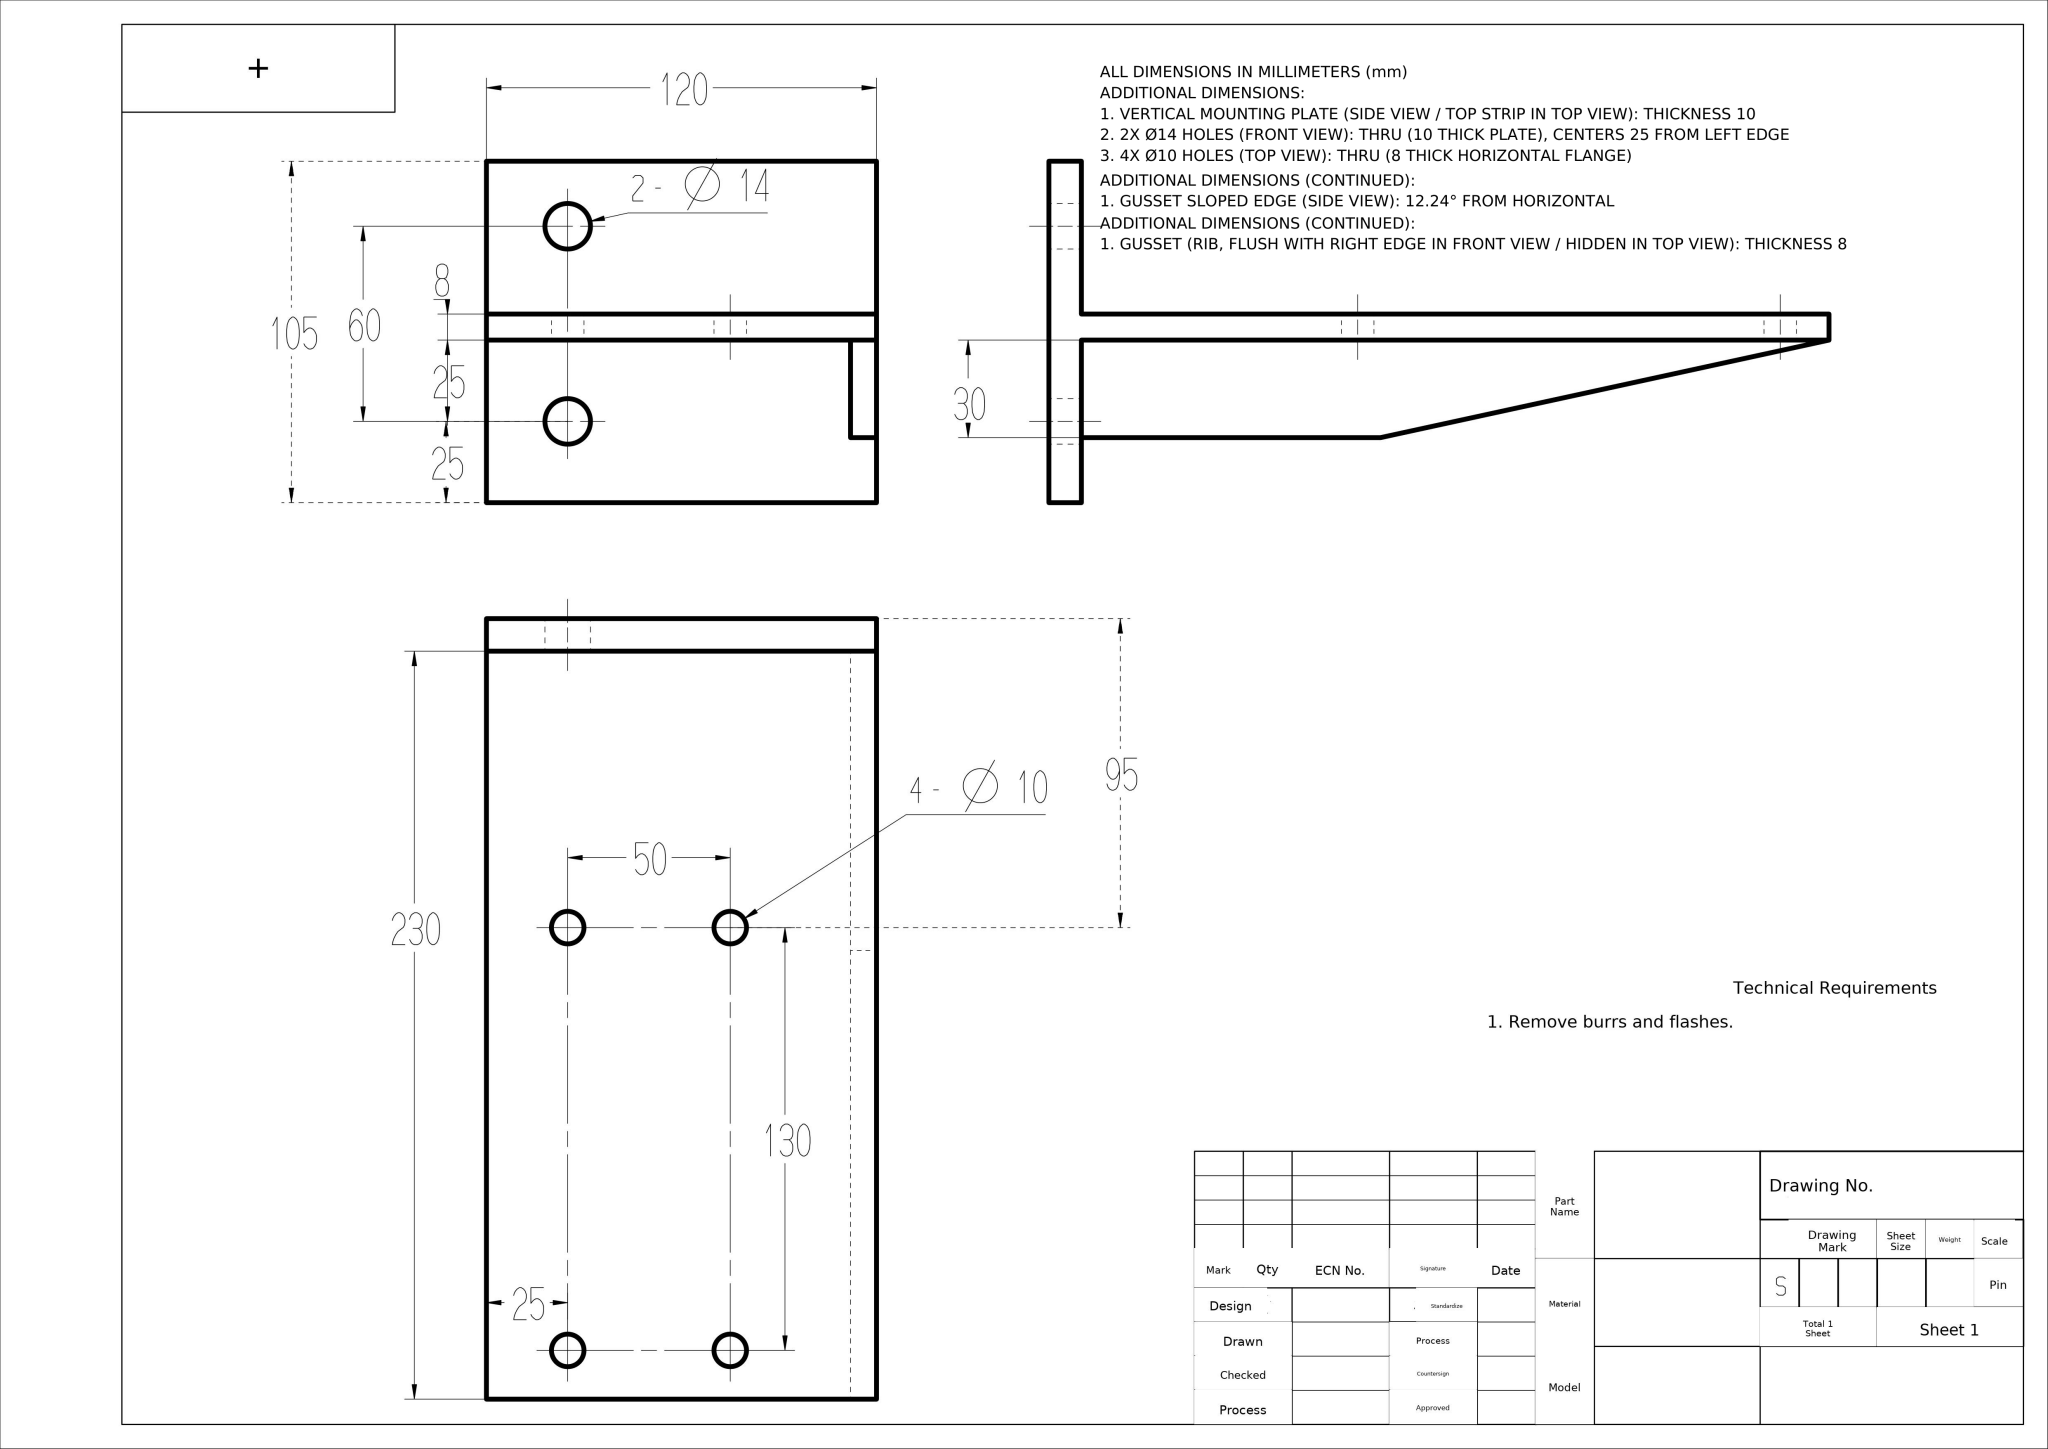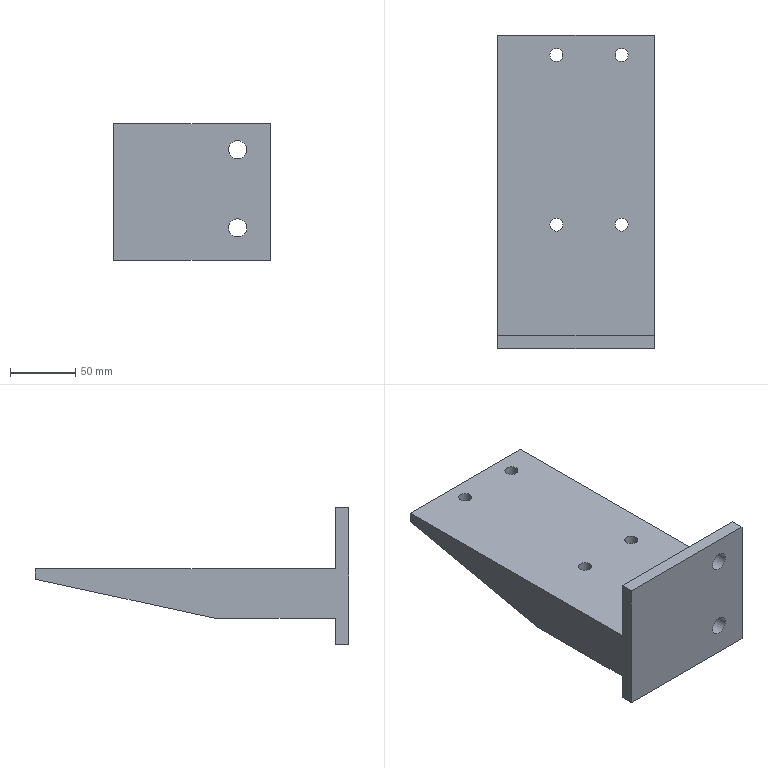Part | NX | mm | 1 solid | 19 faces | box 120 x 240 x 105 mm | volume 379848 mm3 | plane 13 | cylinder 6 | commonest cylinder face diameters 10 x4 14 x2
STEP:
#1=CARTESIAN_POINT('',(0.,0.,0.));
#2=DIRECTION('',(0.,0.,1.));
#3=DIRECTION('',(1.,0.,0.));
#4=AXIS2_PLACEMENT_3D('',#1,#2,#3);
#5=(LENGTH_UNIT()NAMED_UNIT(*)SI_UNIT(.MILLI.,.METRE.));
#6=UNCERTAINTY_MEASURE_WITH_UNIT(LENGTH_MEASURE(0.00002),#5,'','');
#7=(NAMED_UNIT(*)PLANE_ANGLE_UNIT()SI_UNIT($,.RADIAN.));
#8=PLANE_ANGLE_MEASURE_WITH_UNIT(PLANE_ANGLE_MEASURE(0.01745),#7);
#9=DIMENSIONAL_EXPONENTS(0.,0.,0.,0.,0.,0.,0.);
#10=(CONVERSION_BASED_UNIT('',#8)NAMED_UNIT(#9)PLANE_ANGLE_UNIT());
#11=(NAMED_UNIT(*)SI_UNIT($,.STERADIAN.)SOLID_ANGLE_UNIT());
#12=(GEOMETRIC_REPRESENTATION_CONTEXT(3)GLOBAL_UNCERTAINTY_ASSIGNED_CONTEXT((#6))GLOBAL_UNIT_ASSIGNED_CONTEXT((#5,#10,#11))REPRESENTATION_CONTEXT('',''));
#13=SHAPE_REPRESENTATION('',(#4),#12);
#14=CARTESIAN_POINT('',(48.,-142.1,0.));
#15=VERTEX_POINT('',#14);
#16=CARTESIAN_POINT('',(43.,-142.1,0.));
#17=DIRECTION('',(0.,0.,-1.));
#18=DIRECTION('',(1.,0.,0.));
#19=AXIS2_PLACEMENT_3D('',#16,#17,#18);
#20=CIRCLE('',#19,5.);
#21=EDGE_CURVE('',#15,#15,#20,.T.);
#22=ORIENTED_EDGE('',*,*,#21,.F.);
#23=EDGE_LOOP('',(#22));
#24=FACE_BOUND('',#23,.T.);
#25=CARTESIAN_POINT('',(48.,-12.1,0.));
#26=VERTEX_POINT('',#25);
#27=CARTESIAN_POINT('',(43.,-12.1,0.));
#28=DIRECTION('',(0.,0.,1.));
#29=DIRECTION('',(1.,0.,0.));
#30=AXIS2_PLACEMENT_3D('',#27,#28,#29);
#31=CIRCLE('',#30,5.);
#32=EDGE_CURVE('',#26,#26,#31,.T.);
#33=ORIENTED_EDGE('',*,*,#32,.T.);
#34=EDGE_LOOP('',(#33));
#35=FACE_BOUND('',#34,.T.);
#36=CARTESIAN_POINT('',(98.,-142.1,0.));
#37=VERTEX_POINT('',#36);
#38=CARTESIAN_POINT('',(93.,-142.1,0.));
#39=DIRECTION('',(0.,0.,1.));
#40=DIRECTION('',(1.,0.,0.));
#41=AXIS2_PLACEMENT_3D('',#38,#39,#40);
#42=CIRCLE('',#41,5.);
#43=EDGE_CURVE('',#37,#37,#42,.T.);
#44=ORIENTED_EDGE('',*,*,#43,.T.);
#45=EDGE_LOOP('',(#44));
#46=FACE_BOUND('',#45,.T.);
#47=CARTESIAN_POINT('',(98.,-12.1,0.));
#48=VERTEX_POINT('',#47);
#49=CARTESIAN_POINT('',(93.,-12.1,0.));
#50=DIRECTION('',(0.,0.,1.));
#51=DIRECTION('',(1.,0.,0.));
#52=AXIS2_PLACEMENT_3D('',#49,#50,#51);
#53=CIRCLE('',#52,5.);
#54=EDGE_CURVE('',#48,#48,#53,.T.);
#55=ORIENTED_EDGE('',*,*,#54,.T.);
#56=EDGE_LOOP('',(#55));
#57=FACE_BOUND('',#56,.T.);
#58=CARTESIAN_POINT('',(118.,-227.1,0.));
#59=VERTEX_POINT('',#58);
#60=CARTESIAN_POINT('',(6.,-227.1,0.));
#61=VERTEX_POINT('',#60);
#62=CARTESIAN_POINT('',(118.,-227.1,0.));
#63=DIRECTION('',(-1.,-0.,0.));
#64=VECTOR('',#63,1.);
#65=LINE('',#62,#64);
#66=EDGE_CURVE('',#59,#61,#65,.T.);
#67=ORIENTED_EDGE('',*,*,#66,.T.);
#68=CARTESIAN_POINT('',(6.,2.9,0.));
#69=VERTEX_POINT('',#68);
#70=CARTESIAN_POINT('',(6.,-227.1,0.));
#71=DIRECTION('',(0.,1.,0.));
#72=VECTOR('',#71,1.);
#73=LINE('',#70,#72);
#74=EDGE_CURVE('',#61,#69,#73,.T.);
#75=ORIENTED_EDGE('',*,*,#74,.T.);
#76=CARTESIAN_POINT('',(118.,2.9,0.));
#77=VERTEX_POINT('',#76);
#78=CARTESIAN_POINT('',(-2.,2.9,0.));
#79=DIRECTION('',(1.,-0.,0.));
#80=VECTOR('',#79,1.);
#81=LINE('',#78,#80);
#82=EDGE_CURVE('',#69,#77,#81,.T.);
#83=ORIENTED_EDGE('',*,*,#82,.T.);
#84=CARTESIAN_POINT('',(118.,2.9,0.));
#85=DIRECTION('',(0.,-1.,0.));
#86=VECTOR('',#85,1.);
#87=LINE('',#84,#86);
#88=EDGE_CURVE('',#77,#59,#87,.T.);
#89=ORIENTED_EDGE('',*,*,#88,.T.);
#90=EDGE_LOOP('',(#67,#75,#83,#89));
#91=FACE_BOUND('',#90,.T.);
#92=CARTESIAN_POINT('',(0.,0.,0.));
#93=DIRECTION('',(0.,0.,-1.));
#94=DIRECTION('',(-1.,0.,0.));
#95=AXIS2_PLACEMENT_3D('',#92,#93,#94);
#96=PLANE('',#95);
#97=ADVANCED_FACE('',(#24,#35,#46,#57,#91),#96,.T.);
#98=CARTESIAN_POINT('',(-2.,2.9,0.));
#99=VERTEX_POINT('',#98);
#100=CARTESIAN_POINT('',(-2.,2.9,0.));
#101=DIRECTION('',(1.,-0.,0.));
#102=VECTOR('',#101,1.);
#103=LINE('',#100,#102);
#104=EDGE_CURVE('',#99,#69,#103,.T.);
#105=ORIENTED_EDGE('',*,*,#104,.F.);
#106=CARTESIAN_POINT('',(-2.,2.9,8.));
#107=VERTEX_POINT('',#106);
#108=CARTESIAN_POINT('',(-2.,2.9,8.));
#109=DIRECTION('',(0.,0.,-1.));
#110=VECTOR('',#109,1.);
#111=LINE('',#108,#110);
#112=EDGE_CURVE('',#107,#99,#111,.T.);
#113=ORIENTED_EDGE('',*,*,#112,.F.);
#114=CARTESIAN_POINT('',(118.,2.9,8.));
#115=VERTEX_POINT('',#114);
#116=CARTESIAN_POINT('',(-2.,2.9,8.));
#117=DIRECTION('',(1.,-0.,0.));
#118=VECTOR('',#117,1.);
#119=LINE('',#116,#118);
#120=EDGE_CURVE('',#107,#115,#119,.T.);
#121=ORIENTED_EDGE('',*,*,#120,.T.);
#122=CARTESIAN_POINT('',(118.,2.9,8.));
#123=DIRECTION('',(0.,0.,-1.));
#124=VECTOR('',#123,1.);
#125=LINE('',#122,#124);
#126=EDGE_CURVE('',#115,#77,#125,.T.);
#127=ORIENTED_EDGE('',*,*,#126,.T.);
#128=ORIENTED_EDGE('',*,*,#82,.F.);
#129=EDGE_LOOP('',(#105,#113,#121,#127,#128));
#130=FACE_OUTER_BOUND('',#129,.T.);
#131=CARTESIAN_POINT('',(-2.,2.9,8.));
#132=DIRECTION('',(0.,1.,0.));
#133=DIRECTION('',(-1.,0.,0.));
#134=AXIS2_PLACEMENT_3D('',#131,#132,#133);
#135=PLANE('',#134);
#136=ADVANCED_FACE('',(#130),#135,.T.);
#137=ORIENTED_EDGE('',*,*,#88,.F.);
#138=ORIENTED_EDGE('',*,*,#126,.F.);
#139=CARTESIAN_POINT('',(118.,-227.1,8.));
#140=VERTEX_POINT('',#139);
#141=CARTESIAN_POINT('',(118.,2.9,8.));
#142=DIRECTION('',(0.,-1.,0.));
#143=VECTOR('',#142,1.);
#144=LINE('',#141,#143);
#145=EDGE_CURVE('',#115,#140,#144,.T.);
#146=ORIENTED_EDGE('',*,*,#145,.T.);
#147=CARTESIAN_POINT('',(118.,-227.1,55.));
#148=VERTEX_POINT('',#147);
#149=CARTESIAN_POINT('',(118.,-227.1,55.));
#150=DIRECTION('',(0.,0.,1.));
#151=VECTOR('',#150,1.);
#152=LINE('',#149,#151);
#153=EDGE_CURVE('',#140,#148,#152,.T.);
#154=ORIENTED_EDGE('',*,*,#153,.T.);
#155=CARTESIAN_POINT('',(118.,-237.1,55.));
#156=VERTEX_POINT('',#155);
#157=CARTESIAN_POINT('',(118.,-237.1,55.));
#158=DIRECTION('',(0.,-1.,0.));
#159=VECTOR('',#158,1.);
#160=LINE('',#157,#159);
#161=EDGE_CURVE('',#148,#156,#160,.T.);
#162=ORIENTED_EDGE('',*,*,#161,.T.);
#163=CARTESIAN_POINT('',(118.,-237.1,-50.));
#164=VERTEX_POINT('',#163);
#165=CARTESIAN_POINT('',(118.,-237.1,55.));
#166=DIRECTION('',(0.,0.,1.));
#167=VECTOR('',#166,1.);
#168=LINE('',#165,#167);
#169=EDGE_CURVE('',#164,#156,#168,.T.);
#170=ORIENTED_EDGE('',*,*,#169,.F.);
#171=CARTESIAN_POINT('',(118.,-227.1,-50.));
#172=VERTEX_POINT('',#171);
#173=CARTESIAN_POINT('',(118.,-237.1,-50.));
#174=DIRECTION('',(0.,-1.,0.));
#175=VECTOR('',#174,1.);
#176=LINE('',#173,#175);
#177=EDGE_CURVE('',#172,#164,#176,.T.);
#178=ORIENTED_EDGE('',*,*,#177,.F.);
#179=CARTESIAN_POINT('',(118.,-227.1,55.));
#180=DIRECTION('',(0.,0.,1.));
#181=VECTOR('',#180,1.);
#182=LINE('',#179,#181);
#183=EDGE_CURVE('',#172,#59,#182,.T.);
#184=ORIENTED_EDGE('',*,*,#183,.T.);
#185=EDGE_LOOP('',(#137,#138,#146,#154,#162,#170,#178,#184));
#186=FACE_OUTER_BOUND('',#185,.T.);
#187=CARTESIAN_POINT('',(118.,2.9,8.));
#188=DIRECTION('',(1.,0.,0.));
#189=DIRECTION('',(0.,0.,-1.));
#190=AXIS2_PLACEMENT_3D('',#187,#188,#189);
#191=PLANE('',#190);
#192=ADVANCED_FACE('',(#186),#191,.T.);
#193=ORIENTED_EDGE('',*,*,#112,.T.);
#194=CARTESIAN_POINT('',(-2.,-135.1,-30.));
#195=VERTEX_POINT('',#194);
#196=CARTESIAN_POINT('',(-2.,2.9,0.));
#197=DIRECTION('',(-0.,-0.9772,-0.2124));
#198=VECTOR('',#197,1.);
#199=LINE('',#196,#198);
#200=EDGE_CURVE('',#99,#195,#199,.T.);
#201=ORIENTED_EDGE('',*,*,#200,.T.);
#202=CARTESIAN_POINT('',(-2.,-227.1,-30.));
#203=VERTEX_POINT('',#202);
#204=CARTESIAN_POINT('',(-2.,-227.1,-30.));
#205=DIRECTION('',(0.,1.,0.));
#206=VECTOR('',#205,1.);
#207=LINE('',#204,#206);
#208=EDGE_CURVE('',#203,#195,#207,.T.);
#209=ORIENTED_EDGE('',*,*,#208,.F.);
#210=CARTESIAN_POINT('',(-2.,-227.1,-50.));
#211=VERTEX_POINT('',#210);
#212=CARTESIAN_POINT('',(-2.,-227.1,-50.));
#213=DIRECTION('',(-0.,0.,-1.));
#214=VECTOR('',#213,1.);
#215=LINE('',#212,#214);
#216=EDGE_CURVE('',#203,#211,#215,.T.);
#217=ORIENTED_EDGE('',*,*,#216,.T.);
#218=CARTESIAN_POINT('',(-2.,-237.1,-50.));
#219=VERTEX_POINT('',#218);
#220=CARTESIAN_POINT('',(-2.,-237.1,-50.));
#221=DIRECTION('',(0.,-1.,0.));
#222=VECTOR('',#221,1.);
#223=LINE('',#220,#222);
#224=EDGE_CURVE('',#211,#219,#223,.T.);
#225=ORIENTED_EDGE('',*,*,#224,.T.);
#226=CARTESIAN_POINT('',(-2.,-237.1,55.));
#227=VERTEX_POINT('',#226);
#228=CARTESIAN_POINT('',(-2.,-237.1,-50.));
#229=DIRECTION('',(-0.,0.,-1.));
#230=VECTOR('',#229,1.);
#231=LINE('',#228,#230);
#232=EDGE_CURVE('',#227,#219,#231,.T.);
#233=ORIENTED_EDGE('',*,*,#232,.F.);
#234=CARTESIAN_POINT('',(-2.,-227.1,55.));
#235=VERTEX_POINT('',#234);
#236=CARTESIAN_POINT('',(-2.,-237.1,55.));
#237=DIRECTION('',(0.,-1.,0.));
#238=VECTOR('',#237,1.);
#239=LINE('',#236,#238);
#240=EDGE_CURVE('',#235,#227,#239,.T.);
#241=ORIENTED_EDGE('',*,*,#240,.F.);
#242=CARTESIAN_POINT('',(-2.,-227.1,8.));
#243=VERTEX_POINT('',#242);
#244=CARTESIAN_POINT('',(-2.,-227.1,-50.));
#245=DIRECTION('',(-0.,0.,-1.));
#246=VECTOR('',#245,1.);
#247=LINE('',#244,#246);
#248=EDGE_CURVE('',#235,#243,#247,.T.);
#249=ORIENTED_EDGE('',*,*,#248,.T.);
#250=CARTESIAN_POINT('',(-2.,-227.1,8.));
#251=DIRECTION('',(0.,1.,0.));
#252=VECTOR('',#251,1.);
#253=LINE('',#250,#252);
#254=EDGE_CURVE('',#243,#107,#253,.T.);
#255=ORIENTED_EDGE('',*,*,#254,.T.);
#256=EDGE_LOOP('',(#193,#201,#209,#217,#225,#233,#241,#249,#255));
#257=FACE_OUTER_BOUND('',#256,.T.);
#258=CARTESIAN_POINT('',(-2.,-227.1,8.));
#259=DIRECTION('',(-1.,0.,0.));
#260=DIRECTION('',(-0.,-1.,0.));
#261=AXIS2_PLACEMENT_3D('',#258,#259,#260);
#262=PLANE('',#261);
#263=ADVANCED_FACE('',(#257),#262,.T.);
#264=CARTESIAN_POINT('',(48.,-142.1,8.));
#265=VERTEX_POINT('',#264);
#266=CARTESIAN_POINT('',(43.,-142.1,8.));
#267=DIRECTION('',(0.,0.,-1.));
#268=DIRECTION('',(1.,0.,0.));
#269=AXIS2_PLACEMENT_3D('',#266,#267,#268);
#270=CIRCLE('',#269,5.);
#271=EDGE_CURVE('',#265,#265,#270,.T.);
#272=ORIENTED_EDGE('',*,*,#271,.T.);
#273=EDGE_LOOP('',(#272));
#274=FACE_BOUND('',#273,.T.);
#275=CARTESIAN_POINT('',(48.,-12.1,8.));
#276=VERTEX_POINT('',#275);
#277=CARTESIAN_POINT('',(43.,-12.1,8.));
#278=DIRECTION('',(0.,0.,1.));
#279=DIRECTION('',(1.,0.,0.));
#280=AXIS2_PLACEMENT_3D('',#277,#278,#279);
#281=CIRCLE('',#280,5.);
#282=EDGE_CURVE('',#276,#276,#281,.T.);
#283=ORIENTED_EDGE('',*,*,#282,.F.);
#284=EDGE_LOOP('',(#283));
#285=FACE_BOUND('',#284,.T.);
#286=CARTESIAN_POINT('',(98.,-142.1,8.));
#287=VERTEX_POINT('',#286);
#288=CARTESIAN_POINT('',(93.,-142.1,8.));
#289=DIRECTION('',(0.,0.,1.));
#290=DIRECTION('',(1.,0.,0.));
#291=AXIS2_PLACEMENT_3D('',#288,#289,#290);
#292=CIRCLE('',#291,5.);
#293=EDGE_CURVE('',#287,#287,#292,.T.);
#294=ORIENTED_EDGE('',*,*,#293,.F.);
#295=EDGE_LOOP('',(#294));
#296=FACE_BOUND('',#295,.T.);
#297=CARTESIAN_POINT('',(98.,-12.1,8.));
#298=VERTEX_POINT('',#297);
#299=CARTESIAN_POINT('',(93.,-12.1,8.));
#300=DIRECTION('',(0.,0.,1.));
#301=DIRECTION('',(1.,0.,0.));
#302=AXIS2_PLACEMENT_3D('',#299,#300,#301);
#303=CIRCLE('',#302,5.);
#304=EDGE_CURVE('',#298,#298,#303,.T.);
#305=ORIENTED_EDGE('',*,*,#304,.F.);
#306=EDGE_LOOP('',(#305));
#307=FACE_BOUND('',#306,.T.);
#308=ORIENTED_EDGE('',*,*,#120,.F.);
#309=ORIENTED_EDGE('',*,*,#254,.F.);
#310=CARTESIAN_POINT('',(118.,-227.1,8.));
#311=DIRECTION('',(-1.,-0.,0.));
#312=VECTOR('',#311,1.);
#313=LINE('',#310,#312);
#314=EDGE_CURVE('',#140,#243,#313,.T.);
#315=ORIENTED_EDGE('',*,*,#314,.F.);
#316=ORIENTED_EDGE('',*,*,#145,.F.);
#317=EDGE_LOOP('',(#308,#309,#315,#316));
#318=FACE_BOUND('',#317,.T.);
#319=CARTESIAN_POINT('',(0.,0.,8.));
#320=DIRECTION('',(0.,0.,-1.));
#321=DIRECTION('',(-1.,0.,0.));
#322=AXIS2_PLACEMENT_3D('',#319,#320,#321);
#323=PLANE('',#322);
#324=ADVANCED_FACE('',(#274,#285,#296,#307,#318),#323,.F.);
#325=ORIENTED_EDGE('',*,*,#304,.T.);
#326=EDGE_LOOP('',(#325));
#327=FACE_BOUND('',#326,.T.);
#328=ORIENTED_EDGE('',*,*,#54,.F.);
#329=EDGE_LOOP('',(#328));
#330=FACE_BOUND('',#329,.T.);
#331=CARTESIAN_POINT('',(93.,-12.1,8.));
#332=DIRECTION('',(0.,0.,-1.));
#333=DIRECTION('',(-1.,0.,0.));
#334=AXIS2_PLACEMENT_3D('',#331,#332,#333);
#335=CYLINDRICAL_SURFACE('',#334,5.);
#336=ADVANCED_FACE('',(#327,#330),#335,.F.);
#337=ORIENTED_EDGE('',*,*,#293,.T.);
#338=EDGE_LOOP('',(#337));
#339=FACE_BOUND('',#338,.T.);
#340=ORIENTED_EDGE('',*,*,#43,.F.);
#341=EDGE_LOOP('',(#340));
#342=FACE_BOUND('',#341,.T.);
#343=CARTESIAN_POINT('',(93.,-142.1,8.));
#344=DIRECTION('',(0.,0.,-1.));
#345=DIRECTION('',(-1.,0.,0.));
#346=AXIS2_PLACEMENT_3D('',#343,#344,#345);
#347=CYLINDRICAL_SURFACE('',#346,5.);
#348=ADVANCED_FACE('',(#339,#342),#347,.F.);
#349=ORIENTED_EDGE('',*,*,#282,.T.);
#350=EDGE_LOOP('',(#349));
#351=FACE_BOUND('',#350,.T.);
#352=ORIENTED_EDGE('',*,*,#32,.F.);
#353=EDGE_LOOP('',(#352));
#354=FACE_BOUND('',#353,.T.);
#355=CARTESIAN_POINT('',(43.,-12.1,8.));
#356=DIRECTION('',(0.,0.,-1.));
#357=DIRECTION('',(-1.,0.,0.));
#358=AXIS2_PLACEMENT_3D('',#355,#356,#357);
#359=CYLINDRICAL_SURFACE('',#358,5.);
#360=ADVANCED_FACE('',(#351,#354),#359,.F.);
#361=ORIENTED_EDGE('',*,*,#271,.F.);
#362=EDGE_LOOP('',(#361));
#363=FACE_BOUND('',#362,.T.);
#364=ORIENTED_EDGE('',*,*,#21,.T.);
#365=EDGE_LOOP('',(#364));
#366=FACE_BOUND('',#365,.T.);
#367=CARTESIAN_POINT('',(43.,-142.1,8.));
#368=DIRECTION('',(0.,0.,-1.));
#369=DIRECTION('',(-1.,0.,0.));
#370=AXIS2_PLACEMENT_3D('',#367,#368,#369);
#371=CYLINDRICAL_SURFACE('',#370,5.);
#372=ADVANCED_FACE('',(#363,#366),#371,.F.);
#373=CARTESIAN_POINT('',(100.,-227.1,35.));
#374=VERTEX_POINT('',#373);
#375=CARTESIAN_POINT('',(93.,-227.1,35.));
#376=DIRECTION('',(0.,1.,0.));
#377=DIRECTION('',(1.,0.,0.));
#378=AXIS2_PLACEMENT_3D('',#375,#376,#377);
#379=CIRCLE('',#378,7.);
#380=EDGE_CURVE('',#374,#374,#379,.T.);
#381=ORIENTED_EDGE('',*,*,#380,.F.);
#382=EDGE_LOOP('',(#381));
#383=FACE_BOUND('',#382,.T.);
#384=ORIENTED_EDGE('',*,*,#153,.F.);
#385=ORIENTED_EDGE('',*,*,#314,.T.);
#386=ORIENTED_EDGE('',*,*,#248,.F.);
#387=CARTESIAN_POINT('',(-2.,-227.1,55.));
#388=DIRECTION('',(-1.,-0.,0.));
#389=VECTOR('',#388,1.);
#390=LINE('',#387,#389);
#391=EDGE_CURVE('',#148,#235,#390,.T.);
#392=ORIENTED_EDGE('',*,*,#391,.F.);
#393=EDGE_LOOP('',(#384,#385,#386,#392));
#394=FACE_BOUND('',#393,.T.);
#395=CARTESIAN_POINT('',(93.,-227.1,35.));
#396=DIRECTION('',(0.,-1.,0.));
#397=DIRECTION('',(0.,0.,-1.));
#398=AXIS2_PLACEMENT_3D('',#395,#396,#397);
#399=PLANE('',#398);
#400=ADVANCED_FACE('',(#383,#394),#399,.F.);
#401=ORIENTED_EDGE('',*,*,#66,.F.);
#402=ORIENTED_EDGE('',*,*,#183,.F.);
#403=CARTESIAN_POINT('',(118.,-227.1,-50.));
#404=DIRECTION('',(1.,0.,0.));
#405=VECTOR('',#404,1.);
#406=LINE('',#403,#405);
#407=EDGE_CURVE('',#211,#172,#406,.T.);
#408=ORIENTED_EDGE('',*,*,#407,.F.);
#409=ORIENTED_EDGE('',*,*,#216,.F.);
#410=CARTESIAN_POINT('',(6.,-227.1,-30.));
#411=VERTEX_POINT('',#410);
#412=CARTESIAN_POINT('',(6.,-227.1,-30.));
#413=DIRECTION('',(-1.,0.,0.));
#414=VECTOR('',#413,1.);
#415=LINE('',#412,#414);
#416=EDGE_CURVE('',#411,#203,#415,.T.);
#417=ORIENTED_EDGE('',*,*,#416,.F.);
#418=CARTESIAN_POINT('',(6.,-227.1,-50.));
#419=DIRECTION('',(0.,-0.,1.));
#420=VECTOR('',#419,1.);
#421=LINE('',#418,#420);
#422=EDGE_CURVE('',#411,#61,#421,.T.);
#423=ORIENTED_EDGE('',*,*,#422,.T.);
#424=EDGE_LOOP('',(#401,#402,#408,#409,#417,#423));
#425=FACE_BOUND('',#424,.T.);
#426=CARTESIAN_POINT('',(100.,-227.1,-25.));
#427=VERTEX_POINT('',#426);
#428=CARTESIAN_POINT('',(93.,-227.1,-25.));
#429=DIRECTION('',(0.,1.,0.));
#430=DIRECTION('',(1.,0.,0.));
#431=AXIS2_PLACEMENT_3D('',#428,#429,#430);
#432=CIRCLE('',#431,7.);
#433=EDGE_CURVE('',#427,#427,#432,.T.);
#434=ORIENTED_EDGE('',*,*,#433,.F.);
#435=EDGE_LOOP('',(#434));
#436=FACE_BOUND('',#435,.T.);
#437=CARTESIAN_POINT('',(93.,-227.1,35.));
#438=DIRECTION('',(0.,-1.,0.));
#439=DIRECTION('',(0.,0.,-1.));
#440=AXIS2_PLACEMENT_3D('',#437,#438,#439);
#441=PLANE('',#440);
#442=ADVANCED_FACE('',(#425,#436),#441,.F.);
#443=ORIENTED_EDGE('',*,*,#391,.T.);
#444=ORIENTED_EDGE('',*,*,#240,.T.);
#445=CARTESIAN_POINT('',(-2.,-237.1,55.));
#446=DIRECTION('',(-1.,-0.,0.));
#447=VECTOR('',#446,1.);
#448=LINE('',#445,#447);
#449=EDGE_CURVE('',#156,#227,#448,.T.);
#450=ORIENTED_EDGE('',*,*,#449,.F.);
#451=ORIENTED_EDGE('',*,*,#161,.F.);
#452=EDGE_LOOP('',(#443,#444,#450,#451));
#453=FACE_OUTER_BOUND('',#452,.T.);
#454=CARTESIAN_POINT('',(-2.,-237.1,55.));
#455=DIRECTION('',(0.,0.,1.));
#456=DIRECTION('',(1.,0.,-0.));
#457=AXIS2_PLACEMENT_3D('',#454,#455,#456);
#458=PLANE('',#457);
#459=ADVANCED_FACE('',(#453),#458,.T.);
#460=CARTESIAN_POINT('',(100.,-237.1,35.));
#461=VERTEX_POINT('',#460);
#462=CARTESIAN_POINT('',(93.,-237.1,35.));
#463=DIRECTION('',(0.,1.,0.));
#464=DIRECTION('',(1.,0.,0.));
#465=AXIS2_PLACEMENT_3D('',#462,#463,#464);
#466=CIRCLE('',#465,7.);
#467=EDGE_CURVE('',#461,#461,#466,.T.);
#468=ORIENTED_EDGE('',*,*,#467,.F.);
#469=EDGE_LOOP('',(#468));
#470=FACE_BOUND('',#469,.T.);
#471=ORIENTED_EDGE('',*,*,#380,.T.);
#472=EDGE_LOOP('',(#471));
#473=FACE_BOUND('',#472,.T.);
#474=CARTESIAN_POINT('',(93.,-237.1,35.));
#475=DIRECTION('',(0.,1.,0.));
#476=DIRECTION('',(0.,0.,1.));
#477=AXIS2_PLACEMENT_3D('',#474,#475,#476);
#478=CYLINDRICAL_SURFACE('',#477,7.);
#479=ADVANCED_FACE('',(#470,#473),#478,.F.);
#480=ORIENTED_EDGE('',*,*,#407,.T.);
#481=ORIENTED_EDGE('',*,*,#177,.T.);
#482=CARTESIAN_POINT('',(118.,-237.1,-50.));
#483=DIRECTION('',(1.,0.,0.));
#484=VECTOR('',#483,1.);
#485=LINE('',#482,#484);
#486=EDGE_CURVE('',#219,#164,#485,.T.);
#487=ORIENTED_EDGE('',*,*,#486,.F.);
#488=ORIENTED_EDGE('',*,*,#224,.F.);
#489=EDGE_LOOP('',(#480,#481,#487,#488));
#490=FACE_OUTER_BOUND('',#489,.T.);
#491=CARTESIAN_POINT('',(118.,-237.1,-50.));
#492=DIRECTION('',(0.,0.,-1.));
#493=DIRECTION('',(-1.,0.,0.));
#494=AXIS2_PLACEMENT_3D('',#491,#492,#493);
#495=PLANE('',#494);
#496=ADVANCED_FACE('',(#490),#495,.T.);
#497=CARTESIAN_POINT('',(100.,-237.1,-25.));
#498=VERTEX_POINT('',#497);
#499=CARTESIAN_POINT('',(93.,-237.1,-25.));
#500=DIRECTION('',(0.,1.,0.));
#501=DIRECTION('',(1.,0.,0.));
#502=AXIS2_PLACEMENT_3D('',#499,#500,#501);
#503=CIRCLE('',#502,7.);
#504=EDGE_CURVE('',#498,#498,#503,.T.);
#505=ORIENTED_EDGE('',*,*,#504,.F.);
#506=EDGE_LOOP('',(#505));
#507=FACE_BOUND('',#506,.T.);
#508=ORIENTED_EDGE('',*,*,#433,.T.);
#509=EDGE_LOOP('',(#508));
#510=FACE_BOUND('',#509,.T.);
#511=CARTESIAN_POINT('',(93.,-237.1,-25.));
#512=DIRECTION('',(0.,1.,0.));
#513=DIRECTION('',(0.,0.,1.));
#514=AXIS2_PLACEMENT_3D('',#511,#512,#513);
#515=CYLINDRICAL_SURFACE('',#514,7.);
#516=ADVANCED_FACE('',(#507,#510),#515,.F.);
#517=ORIENTED_EDGE('',*,*,#232,.T.);
#518=ORIENTED_EDGE('',*,*,#486,.T.);
#519=ORIENTED_EDGE('',*,*,#169,.T.);
#520=ORIENTED_EDGE('',*,*,#449,.T.);
#521=EDGE_LOOP('',(#517,#518,#519,#520));
#522=FACE_BOUND('',#521,.T.);
#523=ORIENTED_EDGE('',*,*,#467,.T.);
#524=EDGE_LOOP('',(#523));
#525=FACE_BOUND('',#524,.T.);
#526=ORIENTED_EDGE('',*,*,#504,.T.);
#527=EDGE_LOOP('',(#526));
#528=FACE_BOUND('',#527,.T.);
#529=CARTESIAN_POINT('',(93.,-237.1,35.));
#530=DIRECTION('',(0.,-1.,0.));
#531=DIRECTION('',(0.,0.,-1.));
#532=AXIS2_PLACEMENT_3D('',#529,#530,#531);
#533=PLANE('',#532);
#534=ADVANCED_FACE('',(#522,#525,#528),#533,.T.);
#535=CARTESIAN_POINT('',(6.,-135.1,-30.));
#536=VERTEX_POINT('',#535);
#537=CARTESIAN_POINT('',(6.,2.9,0.));
#538=DIRECTION('',(-0.,-0.9772,-0.2124));
#539=VECTOR('',#538,1.);
#540=LINE('',#537,#539);
#541=EDGE_CURVE('',#69,#536,#540,.T.);
#542=ORIENTED_EDGE('',*,*,#541,.T.);
#543=CARTESIAN_POINT('',(6.,-135.1,-30.));
#544=DIRECTION('',(-1.,0.,0.));
#545=VECTOR('',#544,1.);
#546=LINE('',#543,#545);
#547=EDGE_CURVE('',#536,#195,#546,.T.);
#548=ORIENTED_EDGE('',*,*,#547,.T.);
#549=ORIENTED_EDGE('',*,*,#200,.F.);
#550=ORIENTED_EDGE('',*,*,#104,.T.);
#551=EDGE_LOOP('',(#542,#548,#549,#550));
#552=FACE_OUTER_BOUND('',#551,.T.);
#553=CARTESIAN_POINT('',(6.,2.9,0.));
#554=DIRECTION('',(0.,0.2124,-0.9772));
#555=DIRECTION('',(0.,0.9772,0.2124));
#556=AXIS2_PLACEMENT_3D('',#553,#554,#555);
#557=PLANE('',#556);
#558=ADVANCED_FACE('',(#552),#557,.T.);
#559=ORIENTED_EDGE('',*,*,#422,.F.);
#560=CARTESIAN_POINT('',(6.,-227.1,-30.));
#561=DIRECTION('',(0.,1.,0.));
#562=VECTOR('',#561,1.);
#563=LINE('',#560,#562);
#564=EDGE_CURVE('',#411,#536,#563,.T.);
#565=ORIENTED_EDGE('',*,*,#564,.T.);
#566=ORIENTED_EDGE('',*,*,#541,.F.);
#567=ORIENTED_EDGE('',*,*,#74,.F.);
#568=EDGE_LOOP('',(#559,#565,#566,#567));
#569=FACE_OUTER_BOUND('',#568,.T.);
#570=CARTESIAN_POINT('',(6.,0.,0.));
#571=DIRECTION('',(1.,0.,-0.));
#572=DIRECTION('',(-0.,0.,-1.));
#573=AXIS2_PLACEMENT_3D('',#570,#571,#572);
#574=PLANE('',#573);
#575=ADVANCED_FACE('',(#569),#574,.T.);
#576=ORIENTED_EDGE('',*,*,#208,.T.);
#577=ORIENTED_EDGE('',*,*,#547,.F.);
#578=ORIENTED_EDGE('',*,*,#564,.F.);
#579=ORIENTED_EDGE('',*,*,#416,.T.);
#580=EDGE_LOOP('',(#576,#577,#578,#579));
#581=FACE_OUTER_BOUND('',#580,.T.);
#582=CARTESIAN_POINT('',(6.,-227.1,-30.));
#583=DIRECTION('',(0.,0.,1.));
#584=DIRECTION('',(1.,0.,0.));
#585=AXIS2_PLACEMENT_3D('',#582,#583,#584);
#586=PLANE('',#585);
#587=ADVANCED_FACE('',(#581),#586,.F.);
#588=CLOSED_SHELL('',(#97,#136,#192,#263,#324,#336,#348,#360,#372,#400,#442,#459,#479,#496,#516,#534,#558,#575,#587));
#589=MANIFOLD_SOLID_BREP('',#588);
#590=ADVANCED_BREP_SHAPE_REPRESENTATION('',(#589),#12);
#591=SHAPE_REPRESENTATION_RELATIONSHIP('','',#13,#590);
#592=PRESENTATION_LAYER_ASSIGNMENT('','',(#589));
#593=COLOUR_RGB('',1.,0.6,0.);
#594=FILL_AREA_STYLE_COLOUR('',#593);
#595=FILL_AREA_STYLE('',(#594));
#596=SURFACE_STYLE_FILL_AREA(#595);
#597=SURFACE_SIDE_STYLE('',(#596));
#598=SURFACE_STYLE_USAGE(.BOTH.,#597);
#599=PRESENTATION_STYLE_ASSIGNMENT((#598));
#600=STYLED_ITEM('',(#599),#589);
#601=MECHANICAL_DESIGN_GEOMETRIC_PRESENTATION_REPRESENTATION('',(#600),#12);